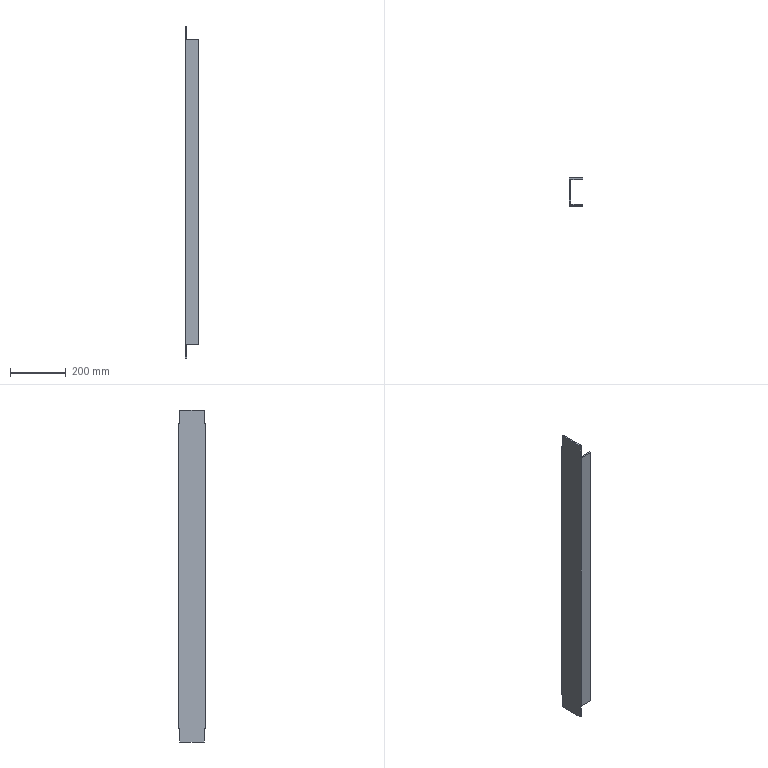Component | SolidWorks | 05TransformerBaseI-1 | 1 solid | 26 faces | box 48 x 100 x 1189 mm | volume 1154519 mm3 | plane 18 | cylinder 8 | commonest cylinder face diameters 12 x8
build123d program:
from build123d import *

# Parameters (mm, degrees)
EXTRUDE_THIN1_DEPTH            = 1189
SKETCH2_W                      = 48
SKETCH2_H                      = 50
CUT_EXTRUDE1_DEPTH             = 5.5
SKETCH3_W                      = 48
SKETCH3_H                      = 50
CUT_EXTRUDE2_DEPTH             = 5.5
F_12_0_12_DIAMETER_HOLE1_D     = 12
F_12_0_12_DIAMETER_HOLE1_DEPTH = 5.5


with BuildPart() as part:
    # Sketch1 → Extrude-Thin1 (new body)
    with BuildSketch(Plane.XY):
        Polygon((48, 0), (0, 0), (0, 100), (48, 100), (48, 94.5), (5.5, 94.5), (5.5, 5.5), (48, 5.5), align=None)
    extrude(amount=EXTRUDE_THIN1_DEPTH)

    # Sketch2 → Cut-Extrude1 (cut)
    with BuildSketch(Plane(origin=(0, 100, 0), x_dir=(1, 0, 0), z_dir=(0, 1, 0))):
        with Locations((24, -1164)):
            Rectangle(SKETCH2_W, SKETCH2_H)
        with Locations((24, -25)):
            Rectangle(SKETCH2_W, SKETCH2_H)
    extrude(amount=-CUT_EXTRUDE1_DEPTH, mode=Mode.SUBTRACT)

    # Sketch3 → Cut-Extrude2 (cut)
    with BuildSketch(Plane.XZ):
        with Locations((24, 25)):
            Rectangle(SKETCH3_W, SKETCH3_H)
        with Locations((24, 1164)):
            Rectangle(SKETCH3_W, SKETCH3_H)
    extrude(amount=-CUT_EXTRUDE2_DEPTH, mode=Mode.SUBTRACT)

    # 12.0 _12_ Diameter Hole1
    with Locations(Plane(origin=(0, 100, 0), x_dir=(-1, 0, 0), z_dir=(0, 1, 0))):
        with Locations((-25, 242.5), (-25, 302.5), (-25, 449.5), (-25, 1109.5)):
            Hole(F_12_0_12_DIAMETER_HOLE1_D / 2, depth=F_12_0_12_DIAMETER_HOLE1_DEPTH)


solid = part.part

# Placed as in the assembly
solid = solid.moved(Location((801.473, -139.54, 42.607), (0, 0, 0)))
STEP:
#1=CARTESIAN_POINT('',(32.538,-1.773,10.988));
#2=VERTEX_POINT('',#1);
#3=CARTESIAN_POINT('',(32.538,-1.773,11.461));
#4=VERTEX_POINT('',#3);
#5=CARTESIAN_POINT('',(32.538,-1.773,11.225));
#6=DIRECTION('',(0.,1.,0.));
#7=DIRECTION('',(0.,0.,1.));
#8=AXIS2_PLACEMENT_3D('',#5,#6,#7);
#9=CIRCLE('',#8,0.2362);
#10=EDGE_CURVE('',#2,#4,#9,.T.);
#11=ORIENTED_EDGE('',*,*,#10,.F.);
#12=CARTESIAN_POINT('',(32.538,-1.557,10.988));
#13=VERTEX_POINT('',#12);
#14=CARTESIAN_POINT('',(32.538,-1.557,10.988));
#15=DIRECTION('',(0.,1.,0.));
#16=VECTOR('',#15,39.37);
#17=LINE('',#14,#16);
#18=EDGE_CURVE('',#2,#13,#17,.T.);
#19=ORIENTED_EDGE('',*,*,#18,.T.);
#20=CARTESIAN_POINT('',(32.538,-1.557,11.461));
#21=VERTEX_POINT('',#20);
#22=CARTESIAN_POINT('',(32.538,-1.557,11.225));
#23=DIRECTION('',(0.,1.,0.));
#24=DIRECTION('',(0.,0.,1.));
#25=AXIS2_PLACEMENT_3D('',#22,#23,#24);
#26=CIRCLE('',#25,0.2362);
#27=EDGE_CURVE('',#13,#21,#26,.T.);
#28=ORIENTED_EDGE('',*,*,#27,.T.);
#29=CARTESIAN_POINT('',(32.538,-1.557,11.461));
#30=DIRECTION('',(0.,1.,0.));
#31=VECTOR('',#30,39.37);
#32=LINE('',#29,#31);
#33=EDGE_CURVE('',#4,#21,#32,.T.);
#34=ORIENTED_EDGE('',*,*,#33,.F.);
#35=EDGE_LOOP('',(#11,#19,#28,#34));
#36=FACE_OUTER_BOUND('',#35,.T.);
#37=CARTESIAN_POINT('',(32.538,-1.557,11.225));
#38=DIRECTION('',(0.,1.,0.));
#39=DIRECTION('',(0.,0.,1.));
#40=AXIS2_PLACEMENT_3D('',#37,#38,#39);
#41=CYLINDRICAL_SURFACE('',#40,0.2362);
#42=ADVANCED_FACE('',(#36),#41,.F.);
#43=CARTESIAN_POINT('',(32.538,-1.773,13.351));
#44=VERTEX_POINT('',#43);
#45=CARTESIAN_POINT('',(32.538,-1.773,13.823));
#46=VERTEX_POINT('',#45);
#47=CARTESIAN_POINT('',(32.538,-1.773,13.587));
#48=DIRECTION('',(0.,1.,0.));
#49=DIRECTION('',(0.,0.,1.));
#50=AXIS2_PLACEMENT_3D('',#47,#48,#49);
#51=CIRCLE('',#50,0.2362);
#52=EDGE_CURVE('',#44,#46,#51,.T.);
#53=ORIENTED_EDGE('',*,*,#52,.F.);
#54=CARTESIAN_POINT('',(32.538,-1.557,13.351));
#55=VERTEX_POINT('',#54);
#56=CARTESIAN_POINT('',(32.538,-1.557,13.351));
#57=DIRECTION('',(0.,1.,0.));
#58=VECTOR('',#57,39.37);
#59=LINE('',#56,#58);
#60=EDGE_CURVE('',#44,#55,#59,.T.);
#61=ORIENTED_EDGE('',*,*,#60,.T.);
#62=CARTESIAN_POINT('',(32.538,-1.557,13.823));
#63=VERTEX_POINT('',#62);
#64=CARTESIAN_POINT('',(32.538,-1.557,13.587));
#65=DIRECTION('',(0.,1.,0.));
#66=DIRECTION('',(0.,0.,1.));
#67=AXIS2_PLACEMENT_3D('',#64,#65,#66);
#68=CIRCLE('',#67,0.2362);
#69=EDGE_CURVE('',#55,#63,#68,.T.);
#70=ORIENTED_EDGE('',*,*,#69,.T.);
#71=CARTESIAN_POINT('',(32.538,-1.557,13.823));
#72=DIRECTION('',(0.,1.,0.));
#73=VECTOR('',#72,39.37);
#74=LINE('',#71,#73);
#75=EDGE_CURVE('',#46,#63,#74,.T.);
#76=ORIENTED_EDGE('',*,*,#75,.F.);
#77=EDGE_LOOP('',(#53,#61,#70,#76));
#78=FACE_OUTER_BOUND('',#77,.T.);
#79=CARTESIAN_POINT('',(32.538,-1.557,13.587));
#80=DIRECTION('',(0.,1.,0.));
#81=DIRECTION('',(0.,0.,1.));
#82=AXIS2_PLACEMENT_3D('',#79,#80,#81);
#83=CYLINDRICAL_SURFACE('',#82,0.2362);
#84=ADVANCED_FACE('',(#78),#83,.F.);
#85=CARTESIAN_POINT('',(32.538,-1.773,19.138));
#86=VERTEX_POINT('',#85);
#87=CARTESIAN_POINT('',(32.538,-1.773,19.611));
#88=VERTEX_POINT('',#87);
#89=CARTESIAN_POINT('',(32.538,-1.773,19.374));
#90=DIRECTION('',(0.,1.,0.));
#91=DIRECTION('',(0.,0.,1.));
#92=AXIS2_PLACEMENT_3D('',#89,#90,#91);
#93=CIRCLE('',#92,0.2362);
#94=EDGE_CURVE('',#86,#88,#93,.T.);
#95=ORIENTED_EDGE('',*,*,#94,.F.);
#96=CARTESIAN_POINT('',(32.538,-1.557,19.138));
#97=VERTEX_POINT('',#96);
#98=CARTESIAN_POINT('',(32.538,-1.557,19.138));
#99=DIRECTION('',(0.,1.,0.));
#100=VECTOR('',#99,39.37);
#101=LINE('',#98,#100);
#102=EDGE_CURVE('',#86,#97,#101,.T.);
#103=ORIENTED_EDGE('',*,*,#102,.T.);
#104=CARTESIAN_POINT('',(32.538,-1.557,19.611));
#105=VERTEX_POINT('',#104);
#106=CARTESIAN_POINT('',(32.538,-1.557,19.374));
#107=DIRECTION('',(0.,1.,0.));
#108=DIRECTION('',(0.,0.,1.));
#109=AXIS2_PLACEMENT_3D('',#106,#107,#108);
#110=CIRCLE('',#109,0.2362);
#111=EDGE_CURVE('',#97,#105,#110,.T.);
#112=ORIENTED_EDGE('',*,*,#111,.T.);
#113=CARTESIAN_POINT('',(32.538,-1.557,19.611));
#114=DIRECTION('',(0.,1.,0.));
#115=VECTOR('',#114,39.37);
#116=LINE('',#113,#115);
#117=EDGE_CURVE('',#88,#105,#116,.T.);
#118=ORIENTED_EDGE('',*,*,#117,.F.);
#119=EDGE_LOOP('',(#95,#103,#112,#118));
#120=FACE_OUTER_BOUND('',#119,.T.);
#121=CARTESIAN_POINT('',(32.538,-1.557,19.374));
#122=DIRECTION('',(0.,1.,0.));
#123=DIRECTION('',(0.,0.,1.));
#124=AXIS2_PLACEMENT_3D('',#121,#122,#123);
#125=CYLINDRICAL_SURFACE('',#124,0.2362);
#126=ADVANCED_FACE('',(#120),#125,.F.);
#127=CARTESIAN_POINT('',(32.538,-1.773,45.122));
#128=VERTEX_POINT('',#127);
#129=CARTESIAN_POINT('',(32.538,-1.773,45.595));
#130=VERTEX_POINT('',#129);
#131=CARTESIAN_POINT('',(32.538,-1.773,45.359));
#132=DIRECTION('',(0.,1.,0.));
#133=DIRECTION('',(0.,0.,1.));
#134=AXIS2_PLACEMENT_3D('',#131,#132,#133);
#135=CIRCLE('',#134,0.2362);
#136=EDGE_CURVE('',#128,#130,#135,.T.);
#137=ORIENTED_EDGE('',*,*,#136,.F.);
#138=CARTESIAN_POINT('',(32.538,-1.557,45.122));
#139=VERTEX_POINT('',#138);
#140=CARTESIAN_POINT('',(32.538,-1.557,45.122));
#141=DIRECTION('',(0.,1.,0.));
#142=VECTOR('',#141,39.37);
#143=LINE('',#140,#142);
#144=EDGE_CURVE('',#128,#139,#143,.T.);
#145=ORIENTED_EDGE('',*,*,#144,.T.);
#146=CARTESIAN_POINT('',(32.538,-1.557,45.595));
#147=VERTEX_POINT('',#146);
#148=CARTESIAN_POINT('',(32.538,-1.557,45.359));
#149=DIRECTION('',(0.,1.,0.));
#150=DIRECTION('',(0.,0.,1.));
#151=AXIS2_PLACEMENT_3D('',#148,#149,#150);
#152=CIRCLE('',#151,0.2362);
#153=EDGE_CURVE('',#139,#147,#152,.T.);
#154=ORIENTED_EDGE('',*,*,#153,.T.);
#155=CARTESIAN_POINT('',(32.538,-1.557,45.595));
#156=DIRECTION('',(0.,1.,0.));
#157=VECTOR('',#156,39.37);
#158=LINE('',#155,#157);
#159=EDGE_CURVE('',#130,#147,#158,.T.);
#160=ORIENTED_EDGE('',*,*,#159,.F.);
#161=EDGE_LOOP('',(#137,#145,#154,#160));
#162=FACE_OUTER_BOUND('',#161,.T.);
#163=CARTESIAN_POINT('',(32.538,-1.557,45.359));
#164=DIRECTION('',(0.,1.,0.));
#165=DIRECTION('',(0.,0.,1.));
#166=AXIS2_PLACEMENT_3D('',#163,#164,#165);
#167=CYLINDRICAL_SURFACE('',#166,0.2362);
#168=ADVANCED_FACE('',(#162),#167,.F.);
#169=CARTESIAN_POINT('',(31.554,-5.277,48.488));
#170=VERTEX_POINT('',#169);
#171=CARTESIAN_POINT('',(31.771,-5.277,48.488));
#172=VERTEX_POINT('',#171);
#173=CARTESIAN_POINT('',(33.444,-5.277,48.488));
#174=DIRECTION('',(1.,-0.,0.));
#175=VECTOR('',#174,39.37);
#176=LINE('',#173,#175);
#177=EDGE_CURVE('',#170,#172,#176,.T.);
#178=ORIENTED_EDGE('',*,*,#177,.T.);
#179=CARTESIAN_POINT('',(31.771,-1.773,48.488));
#180=VERTEX_POINT('',#179);
#181=CARTESIAN_POINT('',(31.771,-5.494,48.488));
#182=DIRECTION('',(0.,1.,0.));
#183=VECTOR('',#182,39.37);
#184=LINE('',#181,#183);
#185=EDGE_CURVE('',#172,#180,#184,.T.);
#186=ORIENTED_EDGE('',*,*,#185,.T.);
#187=CARTESIAN_POINT('',(31.554,-1.773,48.488));
#188=VERTEX_POINT('',#187);
#189=CARTESIAN_POINT('',(33.444,-1.773,48.488));
#190=DIRECTION('',(1.,0.,0.));
#191=VECTOR('',#190,39.37);
#192=LINE('',#189,#191);
#193=EDGE_CURVE('',#188,#180,#192,.T.);
#194=ORIENTED_EDGE('',*,*,#193,.F.);
#195=CARTESIAN_POINT('',(31.554,-5.494,48.488));
#196=DIRECTION('',(0.,1.,0.));
#197=VECTOR('',#196,39.37);
#198=LINE('',#195,#197);
#199=EDGE_CURVE('',#170,#188,#198,.T.);
#200=ORIENTED_EDGE('',*,*,#199,.F.);
#201=EDGE_LOOP('',(#178,#186,#194,#200));
#202=FACE_OUTER_BOUND('',#201,.T.);
#203=CARTESIAN_POINT('',(33.444,-1.773,48.488));
#204=DIRECTION('',(0.,0.,-1.));
#205=DIRECTION('',(-1.,0.,0.));
#206=AXIS2_PLACEMENT_3D('',#203,#204,#205);
#207=PLANE('',#206);
#208=ADVANCED_FACE('',(#202),#207,.F.);
#209=CARTESIAN_POINT('',(31.771,-5.277,1.677));
#210=VERTEX_POINT('',#209);
#211=CARTESIAN_POINT('',(31.771,-1.773,1.677));
#212=VERTEX_POINT('',#211);
#213=CARTESIAN_POINT('',(31.771,-5.494,1.677));
#214=DIRECTION('',(0.,1.,0.));
#215=VECTOR('',#214,39.37);
#216=LINE('',#213,#215);
#217=EDGE_CURVE('',#210,#212,#216,.T.);
#218=ORIENTED_EDGE('',*,*,#217,.F.);
#219=CARTESIAN_POINT('',(31.554,-5.277,1.677));
#220=VERTEX_POINT('',#219);
#221=CARTESIAN_POINT('',(33.444,-5.277,1.677));
#222=DIRECTION('',(-1.,0.,0.));
#223=VECTOR('',#222,39.37);
#224=LINE('',#221,#223);
#225=EDGE_CURVE('',#210,#220,#224,.T.);
#226=ORIENTED_EDGE('',*,*,#225,.T.);
#227=CARTESIAN_POINT('',(31.554,-1.773,1.677));
#228=VERTEX_POINT('',#227);
#229=CARTESIAN_POINT('',(31.554,-5.494,1.677));
#230=DIRECTION('',(0.,1.,0.));
#231=VECTOR('',#230,39.37);
#232=LINE('',#229,#231);
#233=EDGE_CURVE('',#220,#228,#232,.T.);
#234=ORIENTED_EDGE('',*,*,#233,.T.);
#235=CARTESIAN_POINT('',(33.444,-1.773,1.677));
#236=DIRECTION('',(1.,0.,0.));
#237=VECTOR('',#236,39.37);
#238=LINE('',#235,#237);
#239=EDGE_CURVE('',#228,#212,#238,.T.);
#240=ORIENTED_EDGE('',*,*,#239,.T.);
#241=EDGE_LOOP('',(#218,#226,#234,#240));
#242=FACE_OUTER_BOUND('',#241,.T.);
#243=CARTESIAN_POINT('',(33.444,-1.773,1.677));
#244=DIRECTION('',(0.,0.,-1.));
#245=DIRECTION('',(-1.,0.,0.));
#246=AXIS2_PLACEMENT_3D('',#243,#244,#245);
#247=PLANE('',#246);
#248=ADVANCED_FACE('',(#242),#247,.T.);
#249=CARTESIAN_POINT('',(32.538,-1.773,11.225));
#250=DIRECTION('',(0.,1.,0.));
#251=DIRECTION('',(0.,0.,1.));
#252=AXIS2_PLACEMENT_3D('',#249,#250,#251);
#253=CIRCLE('',#252,0.2362);
#254=EDGE_CURVE('',#4,#2,#253,.T.);
#255=ORIENTED_EDGE('',*,*,#254,.T.);
#256=ORIENTED_EDGE('',*,*,#10,.T.);
#257=EDGE_LOOP('',(#255,#256));
#258=FACE_BOUND('',#257,.T.);
#259=CARTESIAN_POINT('',(32.538,-1.773,13.587));
#260=DIRECTION('',(0.,1.,0.));
#261=DIRECTION('',(0.,0.,1.));
#262=AXIS2_PLACEMENT_3D('',#259,#260,#261);
#263=CIRCLE('',#262,0.2362);
#264=EDGE_CURVE('',#46,#44,#263,.T.);
#265=ORIENTED_EDGE('',*,*,#264,.T.);
#266=ORIENTED_EDGE('',*,*,#52,.T.);
#267=EDGE_LOOP('',(#265,#266));
#268=FACE_BOUND('',#267,.T.);
#269=CARTESIAN_POINT('',(32.538,-1.773,19.374));
#270=DIRECTION('',(0.,1.,0.));
#271=DIRECTION('',(0.,0.,1.));
#272=AXIS2_PLACEMENT_3D('',#269,#270,#271);
#273=CIRCLE('',#272,0.2362);
#274=EDGE_CURVE('',#88,#86,#273,.T.);
#275=ORIENTED_EDGE('',*,*,#274,.T.);
#276=ORIENTED_EDGE('',*,*,#94,.T.);
#277=EDGE_LOOP('',(#275,#276));
#278=FACE_BOUND('',#277,.T.);
#279=CARTESIAN_POINT('',(32.538,-1.773,45.359));
#280=DIRECTION('',(0.,1.,0.));
#281=DIRECTION('',(0.,0.,1.));
#282=AXIS2_PLACEMENT_3D('',#279,#280,#281);
#283=CIRCLE('',#282,0.2362);
#284=EDGE_CURVE('',#130,#128,#283,.T.);
#285=ORIENTED_EDGE('',*,*,#284,.T.);
#286=ORIENTED_EDGE('',*,*,#136,.T.);
#287=EDGE_LOOP('',(#285,#286));
#288=FACE_BOUND('',#287,.T.);
#289=CARTESIAN_POINT('',(31.771,-1.773,46.52));
#290=VERTEX_POINT('',#289);
#291=CARTESIAN_POINT('',(31.771,-1.773,3.646));
#292=VERTEX_POINT('',#291);
#293=CARTESIAN_POINT('',(31.771,-1.773,48.488));
#294=DIRECTION('',(0.,0.,-1.));
#295=VECTOR('',#294,39.37);
#296=LINE('',#293,#295);
#297=EDGE_CURVE('',#290,#292,#296,.T.);
#298=ORIENTED_EDGE('',*,*,#297,.T.);
#299=CARTESIAN_POINT('',(33.444,-1.773,3.646));
#300=VERTEX_POINT('',#299);
#301=CARTESIAN_POINT('',(33.444,-1.773,3.646));
#302=DIRECTION('',(-1.,0.,0.));
#303=VECTOR('',#302,39.37);
#304=LINE('',#301,#303);
#305=EDGE_CURVE('',#300,#292,#304,.T.);
#306=ORIENTED_EDGE('',*,*,#305,.F.);
#307=CARTESIAN_POINT('',(33.444,-1.773,46.52));
#308=VERTEX_POINT('',#307);
#309=CARTESIAN_POINT('',(33.444,-1.773,48.488));
#310=DIRECTION('',(0.,0.,-1.));
#311=VECTOR('',#310,39.37);
#312=LINE('',#309,#311);
#313=EDGE_CURVE('',#308,#300,#312,.T.);
#314=ORIENTED_EDGE('',*,*,#313,.F.);
#315=CARTESIAN_POINT('',(33.444,-1.773,46.52));
#316=DIRECTION('',(1.,0.,0.));
#317=VECTOR('',#316,39.37);
#318=LINE('',#315,#317);
#319=EDGE_CURVE('',#290,#308,#318,.T.);
#320=ORIENTED_EDGE('',*,*,#319,.F.);
#321=EDGE_LOOP('',(#298,#306,#314,#320));
#322=FACE_OUTER_BOUND('',#321,.T.);
#323=CARTESIAN_POINT('',(31.554,-1.773,48.488));
#324=DIRECTION('',(0.,1.,0.));
#325=DIRECTION('',(0.,0.,1.));
#326=AXIS2_PLACEMENT_3D('',#323,#324,#325);
#327=PLANE('',#326);
#328=ADVANCED_FACE('',(#258,#268,#278,#288,#322),#327,.F.);
#329=CARTESIAN_POINT('',(33.444,-1.557,3.646));
#330=VERTEX_POINT('',#329);
#331=CARTESIAN_POINT('',(33.444,-4.502,3.646));
#332=DIRECTION('',(0.,1.,0.));
#333=VECTOR('',#332,39.37);
#334=LINE('',#331,#333);
#335=EDGE_CURVE('',#300,#330,#334,.T.);
#336=ORIENTED_EDGE('',*,*,#335,.T.);
#337=CARTESIAN_POINT('',(33.444,-1.557,46.52));
#338=VERTEX_POINT('',#337);
#339=CARTESIAN_POINT('',(33.444,-1.557,48.488));
#340=DIRECTION('',(0.,0.,-1.));
#341=VECTOR('',#340,39.37);
#342=LINE('',#339,#341);
#343=EDGE_CURVE('',#338,#330,#342,.T.);
#344=ORIENTED_EDGE('',*,*,#343,.F.);
#345=CARTESIAN_POINT('',(33.444,-4.502,46.52));
#346=DIRECTION('',(0.,1.,0.));
#347=VECTOR('',#346,39.37);
#348=LINE('',#345,#347);
#349=EDGE_CURVE('',#308,#338,#348,.T.);
#350=ORIENTED_EDGE('',*,*,#349,.F.);
#351=ORIENTED_EDGE('',*,*,#313,.T.);
#352=EDGE_LOOP('',(#336,#344,#350,#351));
#353=FACE_OUTER_BOUND('',#352,.T.);
#354=CARTESIAN_POINT('',(33.444,-1.557,48.488));
#355=DIRECTION('',(1.,0.,0.));
#356=DIRECTION('',(0.,0.,-1.));
#357=AXIS2_PLACEMENT_3D('',#354,#355,#356);
#358=PLANE('',#357);
#359=ADVANCED_FACE('',(#353),#358,.T.);
#360=CARTESIAN_POINT('',(32.538,-1.557,11.225));
#361=DIRECTION('',(0.,1.,0.));
#362=DIRECTION('',(0.,0.,1.));
#363=AXIS2_PLACEMENT_3D('',#360,#361,#362);
#364=CIRCLE('',#363,0.2362);
#365=EDGE_CURVE('',#21,#13,#364,.T.);
#366=ORIENTED_EDGE('',*,*,#365,.F.);
#367=ORIENTED_EDGE('',*,*,#27,.F.);
#368=EDGE_LOOP('',(#366,#367));
#369=FACE_BOUND('',#368,.T.);
#370=CARTESIAN_POINT('',(32.538,-1.557,13.587));
#371=DIRECTION('',(0.,1.,0.));
#372=DIRECTION('',(0.,0.,1.));
#373=AXIS2_PLACEMENT_3D('',#370,#371,#372);
#374=CIRCLE('',#373,0.2362);
#375=EDGE_CURVE('',#63,#55,#374,.T.);
#376=ORIENTED_EDGE('',*,*,#375,.F.);
#377=ORIENTED_EDGE('',*,*,#69,.F.);
#378=EDGE_LOOP('',(#376,#377));
#379=FACE_BOUND('',#378,.T.);
#380=CARTESIAN_POINT('',(32.538,-1.557,19.374));
#381=DIRECTION('',(0.,1.,0.));
#382=DIRECTION('',(0.,0.,1.));
#383=AXIS2_PLACEMENT_3D('',#380,#381,#382);
#384=CIRCLE('',#383,0.2362);
#385=EDGE_CURVE('',#105,#97,#384,.T.);
#386=ORIENTED_EDGE('',*,*,#385,.F.);
#387=ORIENTED_EDGE('',*,*,#111,.F.);
#388=EDGE_LOOP('',(#386,#387));
#389=FACE_BOUND('',#388,.T.);
#390=CARTESIAN_POINT('',(32.538,-1.557,45.359));
#391=DIRECTION('',(0.,1.,0.));
#392=DIRECTION('',(0.,0.,1.));
#393=AXIS2_PLACEMENT_3D('',#390,#391,#392);
#394=CIRCLE('',#393,0.2362);
#395=EDGE_CURVE('',#147,#139,#394,.T.);
#396=ORIENTED_EDGE('',*,*,#395,.F.);
#397=ORIENTED_EDGE('',*,*,#153,.F.);
#398=EDGE_LOOP('',(#396,#397));
#399=FACE_BOUND('',#398,.T.);
#400=CARTESIAN_POINT('',(31.554,-1.557,3.646));
#401=VERTEX_POINT('',#400);
#402=CARTESIAN_POINT('',(33.444,-1.557,3.646));
#403=DIRECTION('',(1.,0.,0.));
#404=VECTOR('',#403,39.37);
#405=LINE('',#402,#404);
#406=EDGE_CURVE('',#401,#330,#405,.T.);
#407=ORIENTED_EDGE('',*,*,#406,.F.);
#408=CARTESIAN_POINT('',(31.554,-1.557,46.52));
#409=VERTEX_POINT('',#408);
#410=CARTESIAN_POINT('',(31.554,-1.557,48.488));
#411=DIRECTION('',(0.,0.,-1.));
#412=VECTOR('',#411,39.37);
#413=LINE('',#410,#412);
#414=EDGE_CURVE('',#409,#401,#413,.T.);
#415=ORIENTED_EDGE('',*,*,#414,.F.);
#416=CARTESIAN_POINT('',(33.444,-1.557,46.52));
#417=DIRECTION('',(-1.,0.,0.));
#418=VECTOR('',#417,39.37);
#419=LINE('',#416,#418);
#420=EDGE_CURVE('',#338,#409,#419,.T.);
#421=ORIENTED_EDGE('',*,*,#420,.F.);
#422=ORIENTED_EDGE('',*,*,#343,.T.);
#423=EDGE_LOOP('',(#407,#415,#421,#422));
#424=FACE_OUTER_BOUND('',#423,.T.);
#425=CARTESIAN_POINT('',(31.554,-1.557,48.488));
#426=DIRECTION('',(0.,1.,0.));
#427=DIRECTION('',(0.,0.,1.));
#428=AXIS2_PLACEMENT_3D('',#425,#426,#427);
#429=PLANE('',#428);
#430=ADVANCED_FACE('',(#369,#379,#389,#399,#424),#429,.T.);
#431=CARTESIAN_POINT('',(31.554,-5.277,46.52));
#432=VERTEX_POINT('',#431);
#433=CARTESIAN_POINT('',(31.554,-5.494,46.52));
#434=VERTEX_POINT('',#433);
#435=CARTESIAN_POINT('',(31.554,-2.548,46.52));
#436=DIRECTION('',(-0.,-1.,0.));
#437=VECTOR('',#436,39.37);
#438=LINE('',#435,#437);
#439=EDGE_CURVE('',#432,#434,#438,.T.);
#440=ORIENTED_EDGE('',*,*,#439,.F.);
#441=CARTESIAN_POINT('',(31.554,-5.277,48.488));
#442=DIRECTION('',(0.,0.,1.));
#443=VECTOR('',#442,39.37);
#444=LINE('',#441,#443);
#445=EDGE_CURVE('',#432,#170,#444,.T.);
#446=ORIENTED_EDGE('',*,*,#445,.T.);
#447=ORIENTED_EDGE('',*,*,#199,.T.);
#448=CARTESIAN_POINT('',(31.554,-1.773,46.52));
#449=VERTEX_POINT('',#448);
#450=CARTESIAN_POINT('',(31.554,-1.773,48.488));
#451=DIRECTION('',(0.,0.,-1.));
#452=VECTOR('',#451,39.37);
#453=LINE('',#450,#452);
#454=EDGE_CURVE('',#188,#449,#453,.T.);
#455=ORIENTED_EDGE('',*,*,#454,.T.);
#456=CARTESIAN_POINT('',(31.554,-4.502,46.52));
#457=DIRECTION('',(0.,1.,0.));
#458=VECTOR('',#457,39.37);
#459=LINE('',#456,#458);
#460=EDGE_CURVE('',#449,#409,#459,.T.);
#461=ORIENTED_EDGE('',*,*,#460,.T.);
#462=ORIENTED_EDGE('',*,*,#414,.T.);
#463=CARTESIAN_POINT('',(31.554,-1.773,3.646));
#464=VERTEX_POINT('',#463);
#465=CARTESIAN_POINT('',(31.554,-4.502,3.646));
#466=DIRECTION('',(0.,1.,0.));
#467=VECTOR('',#466,39.37);
#468=LINE('',#465,#467);
#469=EDGE_CURVE('',#464,#401,#468,.T.);
#470=ORIENTED_EDGE('',*,*,#469,.F.);
#471=CARTESIAN_POINT('',(31.554,-1.773,1.677));
#472=DIRECTION('',(0.,0.,-1.));
#473=VECTOR('',#472,39.37);
#474=LINE('',#471,#473);
#475=EDGE_CURVE('',#464,#228,#474,.T.);
#476=ORIENTED_EDGE('',*,*,#475,.T.);
#477=ORIENTED_EDGE('',*,*,#233,.F.);
#478=CARTESIAN_POINT('',(31.554,-5.277,3.646));
#479=VERTEX_POINT('',#478);
#480=CARTESIAN_POINT('',(31.554,-5.277,1.677));
#481=DIRECTION('',(0.,0.,1.));
#482=VECTOR('',#481,39.37);
#483=LINE('',#480,#482);
#484=EDGE_CURVE('',#220,#479,#483,.T.);
#485=ORIENTED_EDGE('',*,*,#484,.T.);
#486=CARTESIAN_POINT('',(31.554,-5.494,3.646));
#487=VERTEX_POINT('',#486);
#488=CARTESIAN_POINT('',(31.554,-2.548,3.646));
#489=DIRECTION('',(-0.,-1.,0.));
#490=VECTOR('',#489,39.37);
#491=LINE('',#488,#490);
#492=EDGE_CURVE('',#479,#487,#491,.T.);
#493=ORIENTED_EDGE('',*,*,#492,.T.);
#494=CARTESIAN_POINT('',(31.554,-5.494,48.488));
#495=DIRECTION('',(0.,0.,-1.));
#496=VECTOR('',#495,39.37);
#497=LINE('',#494,#496);
#498=EDGE_CURVE('',#434,#487,#497,.T.);
#499=ORIENTED_EDGE('',*,*,#498,.F.);
#500=EDGE_LOOP('',(#440,#446,#447,#455,#461,#462,#470,#476,#477,#485,#493,#499));
#501=FACE_OUTER_BOUND('',#500,.T.);
#502=CARTESIAN_POINT('',(31.554,-5.494,48.488));
#503=DIRECTION('',(-1.,0.,0.));
#504=DIRECTION('',(0.,0.,1.));
#505=AXIS2_PLACEMENT_3D('',#502,#503,#504);
#506=PLANE('',#505);
#507=ADVANCED_FACE('',(#501),#506,.T.);
#508=CARTESIAN_POINT('',(33.444,-5.494,46.52));
#509=VERTEX_POINT('',#508);
#510=CARTESIAN_POINT('',(33.444,-5.494,46.52));
#511=DIRECTION('',(1.,-0.,0.));
#512=VECTOR('',#511,39.37);
#513=LINE('',#510,#512);
#514=EDGE_CURVE('',#434,#509,#513,.T.);
#515=ORIENTED_EDGE('',*,*,#514,.F.);
#516=ORIENTED_EDGE('',*,*,#498,.T.);
#517=CARTESIAN_POINT('',(33.444,-5.494,3.646));
#518=VERTEX_POINT('',#517);
#519=CARTESIAN_POINT('',(33.444,-5.494,3.646));
#520=DIRECTION('',(-1.,0.,0.));
#521=VECTOR('',#520,39.37);
#522=LINE('',#519,#521);
#523=EDGE_CURVE('',#518,#487,#522,.T.);
#524=ORIENTED_EDGE('',*,*,#523,.F.);
#525=CARTESIAN_POINT('',(33.444,-5.494,48.488));
#526=DIRECTION('',(0.,0.,-1.));
#527=VECTOR('',#526,39.37);
#528=LINE('',#525,#527);
#529=EDGE_CURVE('',#509,#518,#528,.T.);
#530=ORIENTED_EDGE('',*,*,#529,.F.);
#531=EDGE_LOOP('',(#515,#516,#524,#530));
#532=FACE_OUTER_BOUND('',#531,.T.);
#533=CARTESIAN_POINT('',(33.444,-5.494,48.488));
#534=DIRECTION('',(-0.,-1.,0.));
#535=DIRECTION('',(1.,-0.,0.));
#536=AXIS2_PLACEMENT_3D('',#533,#534,#535);
#537=PLANE('',#536);
#538=ADVANCED_FACE('',(#532),#537,.T.);
#539=CARTESIAN_POINT('',(33.444,-5.277,46.52));
#540=VERTEX_POINT('',#539);
#541=CARTESIAN_POINT('',(33.444,-2.548,46.52));
#542=DIRECTION('',(-0.,-1.,0.));
#543=VECTOR('',#542,39.37);
#544=LINE('',#541,#543);
#545=EDGE_CURVE('',#540,#509,#544,.T.);
#546=ORIENTED_EDGE('',*,*,#545,.T.);
#547=ORIENTED_EDGE('',*,*,#529,.T.);
#548=CARTESIAN_POINT('',(33.444,-5.277,3.646));
#549=VERTEX_POINT('',#548);
#550=CARTESIAN_POINT('',(33.444,-2.548,3.646));
#551=DIRECTION('',(-0.,-1.,0.));
#552=VECTOR('',#551,39.37);
#553=LINE('',#550,#552);
#554=EDGE_CURVE('',#549,#518,#553,.T.);
#555=ORIENTED_EDGE('',*,*,#554,.F.);
#556=CARTESIAN_POINT('',(33.444,-5.277,48.488));
#557=DIRECTION('',(0.,0.,-1.));
#558=VECTOR('',#557,39.37);
#559=LINE('',#556,#558);
#560=EDGE_CURVE('',#540,#549,#559,.T.);
#561=ORIENTED_EDGE('',*,*,#560,.F.);
#562=EDGE_LOOP('',(#546,#547,#555,#561));
#563=FACE_OUTER_BOUND('',#562,.T.);
#564=CARTESIAN_POINT('',(33.444,-5.277,48.488));
#565=DIRECTION('',(1.,0.,0.));
#566=DIRECTION('',(0.,0.,-1.));
#567=AXIS2_PLACEMENT_3D('',#564,#565,#566);
#568=PLANE('',#567);
#569=ADVANCED_FACE('',(#563),#568,.T.);
#570=CARTESIAN_POINT('',(31.771,-5.277,46.52));
#571=VERTEX_POINT('',#570);
#572=CARTESIAN_POINT('',(31.771,-5.277,3.646));
#573=VERTEX_POINT('',#572);
#574=CARTESIAN_POINT('',(31.771,-5.277,48.488));
#575=DIRECTION('',(0.,0.,-1.));
#576=VECTOR('',#575,39.37);
#577=LINE('',#574,#576);
#578=EDGE_CURVE('',#571,#573,#577,.T.);
#579=ORIENTED_EDGE('',*,*,#578,.F.);
#580=CARTESIAN_POINT('',(33.444,-5.277,46.52));
#581=DIRECTION('',(-1.,0.,0.));
#582=VECTOR('',#581,39.37);
#583=LINE('',#580,#582);
#584=EDGE_CURVE('',#540,#571,#583,.T.);
#585=ORIENTED_EDGE('',*,*,#584,.F.);
#586=ORIENTED_EDGE('',*,*,#560,.T.);
#587=CARTESIAN_POINT('',(33.444,-5.277,3.646));
#588=DIRECTION('',(1.,-0.,0.));
#589=VECTOR('',#588,39.37);
#590=LINE('',#587,#589);
#591=EDGE_CURVE('',#573,#549,#590,.T.);
#592=ORIENTED_EDGE('',*,*,#591,.F.);
#593=EDGE_LOOP('',(#579,#585,#586,#592));
#594=FACE_OUTER_BOUND('',#593,.T.);
#595=CARTESIAN_POINT('',(33.444,-5.277,48.488));
#596=DIRECTION('',(-0.,-1.,0.));
#597=DIRECTION('',(1.,-0.,0.));
#598=AXIS2_PLACEMENT_3D('',#595,#596,#597);
#599=PLANE('',#598);
#600=ADVANCED_FACE('',(#594),#599,.F.);
#601=ORIENTED_EDGE('',*,*,#217,.T.);
#602=CARTESIAN_POINT('',(31.771,-1.773,48.488));
#603=DIRECTION('',(0.,0.,-1.));
#604=VECTOR('',#603,39.37);
#605=LINE('',#602,#604);
#606=EDGE_CURVE('',#292,#212,#605,.T.);
#607=ORIENTED_EDGE('',*,*,#606,.F.);
#608=ORIENTED_EDGE('',*,*,#297,.F.);
#609=CARTESIAN_POINT('',(31.771,-1.773,48.488));
#610=DIRECTION('',(0.,0.,-1.));
#611=VECTOR('',#610,39.37);
#612=LINE('',#609,#611);
#613=EDGE_CURVE('',#180,#290,#612,.T.);
#614=ORIENTED_EDGE('',*,*,#613,.F.);
#615=ORIENTED_EDGE('',*,*,#185,.F.);
#616=CARTESIAN_POINT('',(31.771,-5.277,48.488));
#617=DIRECTION('',(0.,0.,-1.));
#618=VECTOR('',#617,39.37);
#619=LINE('',#616,#618);
#620=EDGE_CURVE('',#172,#571,#619,.T.);
#621=ORIENTED_EDGE('',*,*,#620,.T.);
#622=ORIENTED_EDGE('',*,*,#578,.T.);
#623=CARTESIAN_POINT('',(31.771,-5.277,48.488));
#624=DIRECTION('',(0.,0.,-1.));
#625=VECTOR('',#624,39.37);
#626=LINE('',#623,#625);
#627=EDGE_CURVE('',#573,#210,#626,.T.);
#628=ORIENTED_EDGE('',*,*,#627,.T.);
#629=EDGE_LOOP('',(#601,#607,#608,#614,#615,#621,#622,#628));
#630=FACE_OUTER_BOUND('',#629,.T.);
#631=CARTESIAN_POINT('',(31.771,-5.494,48.488));
#632=DIRECTION('',(-1.,0.,0.));
#633=DIRECTION('',(0.,0.,1.));
#634=AXIS2_PLACEMENT_3D('',#631,#632,#633);
#635=PLANE('',#634);
#636=ADVANCED_FACE('',(#630),#635,.F.);
#637=ORIENTED_EDGE('',*,*,#613,.T.);
#638=CARTESIAN_POINT('',(33.444,-1.773,46.52));
#639=DIRECTION('',(1.,0.,0.));
#640=VECTOR('',#639,39.37);
#641=LINE('',#638,#640);
#642=EDGE_CURVE('',#449,#290,#641,.T.);
#643=ORIENTED_EDGE('',*,*,#642,.F.);
#644=ORIENTED_EDGE('',*,*,#454,.F.);
#645=ORIENTED_EDGE('',*,*,#193,.T.);
#646=EDGE_LOOP('',(#637,#643,#644,#645));
#647=FACE_OUTER_BOUND('',#646,.T.);
#648=CARTESIAN_POINT('',(31.554,-1.773,48.488));
#649=DIRECTION('',(0.,1.,0.));
#650=DIRECTION('',(0.,0.,1.));
#651=AXIS2_PLACEMENT_3D('',#648,#649,#650);
#652=PLANE('',#651);
#653=ADVANCED_FACE('',(#647),#652,.T.);
#654=ORIENTED_EDGE('',*,*,#642,.T.);
#655=ORIENTED_EDGE('',*,*,#319,.T.);
#656=ORIENTED_EDGE('',*,*,#349,.T.);
#657=ORIENTED_EDGE('',*,*,#420,.T.);
#658=ORIENTED_EDGE('',*,*,#460,.F.);
#659=EDGE_LOOP('',(#654,#655,#656,#657,#658));
#660=FACE_OUTER_BOUND('',#659,.T.);
#661=CARTESIAN_POINT('',(33.444,-4.502,46.52));
#662=DIRECTION('',(0.,0.,-1.));
#663=DIRECTION('',(-1.,0.,0.));
#664=AXIS2_PLACEMENT_3D('',#661,#662,#663);
#665=PLANE('',#664);
#666=ADVANCED_FACE('',(#660),#665,.F.);
#667=ORIENTED_EDGE('',*,*,#606,.T.);
#668=ORIENTED_EDGE('',*,*,#239,.F.);
#669=ORIENTED_EDGE('',*,*,#475,.F.);
#670=CARTESIAN_POINT('',(33.444,-1.773,3.646));
#671=DIRECTION('',(-1.,0.,0.));
#672=VECTOR('',#671,39.37);
#673=LINE('',#670,#672);
#674=EDGE_CURVE('',#292,#464,#673,.T.);
#675=ORIENTED_EDGE('',*,*,#674,.F.);
#676=EDGE_LOOP('',(#667,#668,#669,#675));
#677=FACE_OUTER_BOUND('',#676,.T.);
#678=CARTESIAN_POINT('',(31.554,-1.773,48.488));
#679=DIRECTION('',(0.,1.,0.));
#680=DIRECTION('',(0.,0.,1.));
#681=AXIS2_PLACEMENT_3D('',#678,#679,#680);
#682=PLANE('',#681);
#683=ADVANCED_FACE('',(#677),#682,.T.);
#684=ORIENTED_EDGE('',*,*,#305,.T.);
#685=ORIENTED_EDGE('',*,*,#674,.T.);
#686=ORIENTED_EDGE('',*,*,#469,.T.);
#687=ORIENTED_EDGE('',*,*,#406,.T.);
#688=ORIENTED_EDGE('',*,*,#335,.F.);
#689=EDGE_LOOP('',(#684,#685,#686,#687,#688));
#690=FACE_OUTER_BOUND('',#689,.T.);
#691=CARTESIAN_POINT('',(33.444,-4.502,3.646));
#692=DIRECTION('',(0.,0.,1.));
#693=DIRECTION('',(1.,0.,0.));
#694=AXIS2_PLACEMENT_3D('',#691,#692,#693);
#695=PLANE('',#694);
#696=ADVANCED_FACE('',(#690),#695,.F.);
#697=ORIENTED_EDGE('',*,*,#627,.F.);
#698=CARTESIAN_POINT('',(33.444,-5.277,3.646));
#699=DIRECTION('',(1.,-0.,0.));
#700=VECTOR('',#699,39.37);
#701=LINE('',#698,#700);
#702=EDGE_CURVE('',#479,#573,#701,.T.);
#703=ORIENTED_EDGE('',*,*,#702,.F.);
#704=ORIENTED_EDGE('',*,*,#484,.F.);
#705=ORIENTED_EDGE('',*,*,#225,.F.);
#706=EDGE_LOOP('',(#697,#703,#704,#705));
#707=FACE_OUTER_BOUND('',#706,.T.);
#708=CARTESIAN_POINT('',(33.444,-5.277,48.488));
#709=DIRECTION('',(-0.,-1.,0.));
#710=DIRECTION('',(1.,-0.,0.));
#711=AXIS2_PLACEMENT_3D('',#708,#709,#710);
#712=PLANE('',#711);
#713=ADVANCED_FACE('',(#707),#712,.T.);
#714=ORIENTED_EDGE('',*,*,#702,.T.);
#715=ORIENTED_EDGE('',*,*,#591,.T.);
#716=ORIENTED_EDGE('',*,*,#554,.T.);
#717=ORIENTED_EDGE('',*,*,#523,.T.);
#718=ORIENTED_EDGE('',*,*,#492,.F.);
#719=EDGE_LOOP('',(#714,#715,#716,#717,#718));
#720=FACE_OUTER_BOUND('',#719,.T.);
#721=CARTESIAN_POINT('',(33.444,-2.548,3.646));
#722=DIRECTION('',(0.,0.,1.));
#723=DIRECTION('',(1.,0.,0.));
#724=AXIS2_PLACEMENT_3D('',#721,#722,#723);
#725=PLANE('',#724);
#726=ADVANCED_FACE('',(#720),#725,.F.);
#727=ORIENTED_EDGE('',*,*,#620,.F.);
#728=ORIENTED_EDGE('',*,*,#177,.F.);
#729=ORIENTED_EDGE('',*,*,#445,.F.);
#730=CARTESIAN_POINT('',(33.444,-5.277,46.52));
#731=DIRECTION('',(-1.,0.,0.));
#732=VECTOR('',#731,39.37);
#733=LINE('',#730,#732);
#734=EDGE_CURVE('',#571,#432,#733,.T.);
#735=ORIENTED_EDGE('',*,*,#734,.F.);
#736=EDGE_LOOP('',(#727,#728,#729,#735));
#737=FACE_OUTER_BOUND('',#736,.T.);
#738=CARTESIAN_POINT('',(33.444,-5.277,48.488));
#739=DIRECTION('',(-0.,-1.,0.));
#740=DIRECTION('',(1.,-0.,0.));
#741=AXIS2_PLACEMENT_3D('',#738,#739,#740);
#742=PLANE('',#741);
#743=ADVANCED_FACE('',(#737),#742,.T.);
#744=ORIENTED_EDGE('',*,*,#584,.T.);
#745=ORIENTED_EDGE('',*,*,#734,.T.);
#746=ORIENTED_EDGE('',*,*,#439,.T.);
#747=ORIENTED_EDGE('',*,*,#514,.T.);
#748=ORIENTED_EDGE('',*,*,#545,.F.);
#749=EDGE_LOOP('',(#744,#745,#746,#747,#748));
#750=FACE_OUTER_BOUND('',#749,.T.);
#751=CARTESIAN_POINT('',(33.444,-2.548,46.52));
#752=DIRECTION('',(0.,0.,-1.));
#753=DIRECTION('',(-1.,0.,0.));
#754=AXIS2_PLACEMENT_3D('',#751,#752,#753);
#755=PLANE('',#754);
#756=ADVANCED_FACE('',(#750),#755,.F.);
#757=ORIENTED_EDGE('',*,*,#144,.F.);
#758=ORIENTED_EDGE('',*,*,#284,.F.);
#759=ORIENTED_EDGE('',*,*,#159,.T.);
#760=ORIENTED_EDGE('',*,*,#395,.T.);
#761=EDGE_LOOP('',(#757,#758,#759,#760));
#762=FACE_OUTER_BOUND('',#761,.T.);
#763=CARTESIAN_POINT('',(32.538,-1.557,45.359));
#764=DIRECTION('',(0.,1.,0.));
#765=DIRECTION('',(0.,0.,1.));
#766=AXIS2_PLACEMENT_3D('',#763,#764,#765);
#767=CYLINDRICAL_SURFACE('',#766,0.2362);
#768=ADVANCED_FACE('',(#762),#767,.F.);
#769=ORIENTED_EDGE('',*,*,#102,.F.);
#770=ORIENTED_EDGE('',*,*,#274,.F.);
#771=ORIENTED_EDGE('',*,*,#117,.T.);
#772=ORIENTED_EDGE('',*,*,#385,.T.);
#773=EDGE_LOOP('',(#769,#770,#771,#772));
#774=FACE_OUTER_BOUND('',#773,.T.);
#775=CARTESIAN_POINT('',(32.538,-1.557,19.374));
#776=DIRECTION('',(0.,1.,0.));
#777=DIRECTION('',(0.,0.,1.));
#778=AXIS2_PLACEMENT_3D('',#775,#776,#777);
#779=CYLINDRICAL_SURFACE('',#778,0.2362);
#780=ADVANCED_FACE('',(#774),#779,.F.);
#781=ORIENTED_EDGE('',*,*,#60,.F.);
#782=ORIENTED_EDGE('',*,*,#264,.F.);
#783=ORIENTED_EDGE('',*,*,#75,.T.);
#784=ORIENTED_EDGE('',*,*,#375,.T.);
#785=EDGE_LOOP('',(#781,#782,#783,#784));
#786=FACE_OUTER_BOUND('',#785,.T.);
#787=CARTESIAN_POINT('',(32.538,-1.557,13.587));
#788=DIRECTION('',(0.,1.,0.));
#789=DIRECTION('',(0.,0.,1.));
#790=AXIS2_PLACEMENT_3D('',#787,#788,#789);
#791=CYLINDRICAL_SURFACE('',#790,0.2362);
#792=ADVANCED_FACE('',(#786),#791,.F.);
#793=ORIENTED_EDGE('',*,*,#18,.F.);
#794=ORIENTED_EDGE('',*,*,#254,.F.);
#795=ORIENTED_EDGE('',*,*,#33,.T.);
#796=ORIENTED_EDGE('',*,*,#365,.T.);
#797=EDGE_LOOP('',(#793,#794,#795,#796));
#798=FACE_OUTER_BOUND('',#797,.T.);
#799=CARTESIAN_POINT('',(32.538,-1.557,11.225));
#800=DIRECTION('',(0.,1.,0.));
#801=DIRECTION('',(0.,0.,1.));
#802=AXIS2_PLACEMENT_3D('',#799,#800,#801);
#803=CYLINDRICAL_SURFACE('',#802,0.2362);
#804=ADVANCED_FACE('',(#798),#803,.F.);
#805=CLOSED_SHELL('',(#42,#84,#126,#168,#208,#248,#328,#359,#430,#507,#538,#569,#600,#636,#653,#666,#683,#696,#713,#726,#743,#756,#768,#780,#792,#804));
#806=MANIFOLD_SOLID_BREP('',#805);
#807=CARTESIAN_POINT('',(0.,0.,0.));
#808=DIRECTION('',(0.,0.,1.));
#809=DIRECTION('',(1.,0.,0.));
#810=AXIS2_PLACEMENT_3D('',#807,#808,#809);
#811=(LENGTH_UNIT()NAMED_UNIT(*)SI_UNIT($,.METRE.));
#812=LENGTH_MEASURE_WITH_UNIT(LENGTH_MEASURE(0.0254),#811);
#813=DIMENSIONAL_EXPONENTS(1.,0.,0.,0.,0.,0.,0.);
#814=(CONVERSION_BASED_UNIT('',#812)LENGTH_UNIT()NAMED_UNIT(#813));
#815=UNCERTAINTY_MEASURE_WITH_UNIT(LENGTH_MEASURE(0.00001),#814,'','');
#816=(NAMED_UNIT(*)PLANE_ANGLE_UNIT()SI_UNIT($,.RADIAN.));
#817=(NAMED_UNIT(*)SI_UNIT($,.STERADIAN.)SOLID_ANGLE_UNIT());
#818=(GEOMETRIC_REPRESENTATION_CONTEXT(3)GLOBAL_UNCERTAINTY_ASSIGNED_CONTEXT((#815))GLOBAL_UNIT_ASSIGNED_CONTEXT((#814,#816,#817))REPRESENTATION_CONTEXT('',''));
#819=ADVANCED_BREP_SHAPE_REPRESENTATION('',(#806,#810),#818);
#820=COLOUR_RGB('',0.7922,0.8196,0.9333);
#821=FILL_AREA_STYLE_COLOUR('',#820);
#822=FILL_AREA_STYLE('',(#821));
#823=SURFACE_STYLE_FILL_AREA(#822);
#824=SURFACE_SIDE_STYLE('',(#823));
#825=SURFACE_STYLE_USAGE(.BOTH.,#824);
#826=PRESENTATION_STYLE_ASSIGNMENT((#825));
#827=STYLED_ITEM('',(#826),#806);
#828=PRESENTATION_LAYER_ASSIGNMENT('','',(#827));
#829=(LENGTH_UNIT()NAMED_UNIT(*)SI_UNIT($,.METRE.));
#830=LENGTH_MEASURE_WITH_UNIT(LENGTH_MEASURE(0.0254),#829);
#831=DIMENSIONAL_EXPONENTS(1.,0.,0.,0.,0.,0.,0.);
#832=(CONVERSION_BASED_UNIT('',#830)LENGTH_UNIT()NAMED_UNIT(#831));
#833=UNCERTAINTY_MEASURE_WITH_UNIT(LENGTH_MEASURE(0.00001),#832,'','');
#834=(NAMED_UNIT(*)PLANE_ANGLE_UNIT()SI_UNIT($,.RADIAN.));
#835=(NAMED_UNIT(*)SI_UNIT($,.STERADIAN.)SOLID_ANGLE_UNIT());
#836=(GEOMETRIC_REPRESENTATION_CONTEXT(3)GLOBAL_UNCERTAINTY_ASSIGNED_CONTEXT((#833))GLOBAL_UNIT_ASSIGNED_CONTEXT((#832,#834,#835))REPRESENTATION_CONTEXT('',''));
#837=MECHANICAL_DESIGN_GEOMETRIC_PRESENTATION_REPRESENTATION('',(#827),#836);